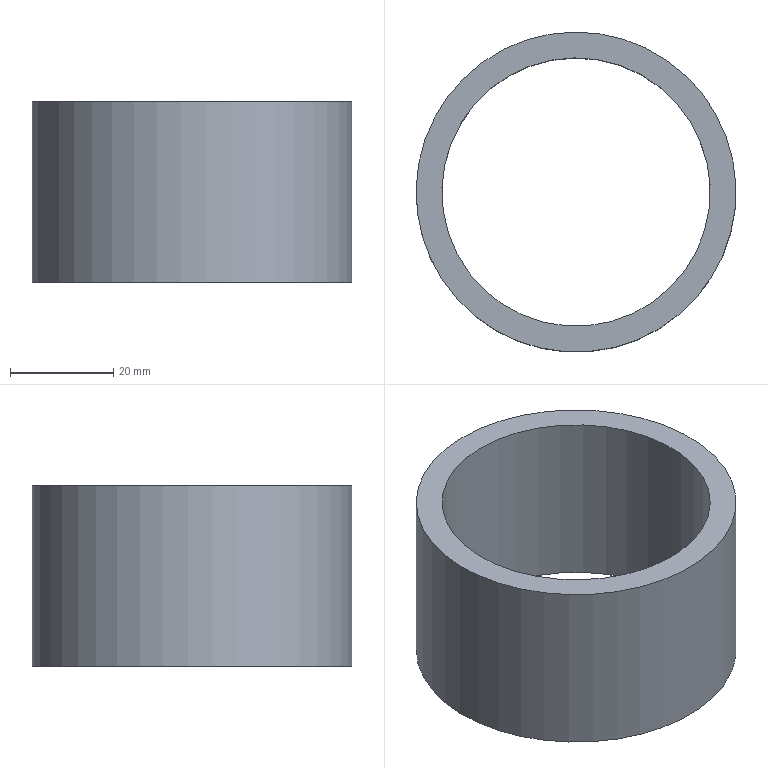Component | NX | CT-ZHOU5-TAOTONG1 | 1 solid | 4 faces | box 62 x 62 x 35 mm | volume 31337 mm3 | cylinder 2 | plane 2 | commonest cylinder face diameters 62 x1 52 x1
STEP:
#1=CARTESIAN_POINT('',(0.,0.,0.));
#2=DIRECTION('',(0.,0.,1.));
#3=DIRECTION('',(1.,0.,0.));
#4=AXIS2_PLACEMENT_3D('',#1,#2,#3);
#5=CARTESIAN_POINT('',(11.875,-28.636,-76.));
#6=VERTEX_POINT('',#5);
#7=CARTESIAN_POINT('',(0.,-0.,-76.));
#8=DIRECTION('',(0.,0.,-1.));
#9=DIRECTION('',(0.383,-0.9237,0.));
#10=AXIS2_PLACEMENT_3D('',#7,#8,#9);
#11=CIRCLE('',#10,31.);
#12=CARTESIAN_POINT('',(0.,-0.,-76.));
#13=DIRECTION('',(0.,0.,1.));
#14=DIRECTION('',(-0.9237,-0.383,0.));
#15=AXIS2_PLACEMENT_3D('',#12,#13,#14);
#16=CYLINDRICAL_SURFACE('',#15,31.);
#17=CARTESIAN_POINT('',(7.854,0.));
#18=DIRECTION('',(-1.,0.));
#19=VECTOR('',#18,1.);
#20=LINE('',#17,#19);
#21=(GEOMETRIC_REPRESENTATION_CONTEXT(2)PARAMETRIC_REPRESENTATION_CONTEXT()REPRESENTATION_CONTEXT('',''));
#22=DEFINITIONAL_REPRESENTATION('',(#20),#21);
#23=PCURVE('',#16,#22);
#24=CARTESIAN_POINT('',(0.,-0.,-76.));
#25=DIRECTION('',(0.,0.,-1.));
#26=DIRECTION('',(0.9237,0.383,0.));
#27=AXIS2_PLACEMENT_3D('',#24,#25,#26);
#28=PLANE('',#27);
#29=CARTESIAN_POINT('',(0.,0.));
#30=DIRECTION('',(0.,1.));
#31=AXIS2_PLACEMENT_2D('',#29,#30);
#32=CIRCLE('',#31,31.);
#33=(GEOMETRIC_REPRESENTATION_CONTEXT(2)PARAMETRIC_REPRESENTATION_CONTEXT()REPRESENTATION_CONTEXT('',''));
#34=DEFINITIONAL_REPRESENTATION('',(#32),#33);
#35=PCURVE('',#28,#34);
#36=SURFACE_CURVE('',#11,(#23,#35),.PCURVE_S1.);
#37=EDGE_CURVE('',#6,#6,#36,.T.);
#38=ORIENTED_EDGE('',*,*,#37,.F.);
#39=CARTESIAN_POINT('',(11.875,-28.636,-41.));
#40=VERTEX_POINT('',#39);
#41=CARTESIAN_POINT('',(11.875,-28.636,-76.));
#42=CARTESIAN_POINT('',(11.875,-28.636,-41.));
#43=B_SPLINE_CURVE_WITH_KNOTS('',1,(#41,#42),.UNSPECIFIED.,.F.,.F.,(2,2),(0.,35.),.PIECEWISE_BEZIER_KNOTS.);
#44=CARTESIAN_POINT('',(7.854,0.));
#45=DIRECTION('',(0.,1.));
#46=VECTOR('',#45,1.);
#47=LINE('',#44,#46);
#48=(GEOMETRIC_REPRESENTATION_CONTEXT(2)PARAMETRIC_REPRESENTATION_CONTEXT()REPRESENTATION_CONTEXT('',''));
#49=DEFINITIONAL_REPRESENTATION('',(#47),#48);
#50=PCURVE('',#16,#49);
#51=CARTESIAN_POINT('',(1.571,0.));
#52=DIRECTION('',(0.,1.));
#53=VECTOR('',#52,1.);
#54=LINE('',#51,#53);
#55=(GEOMETRIC_REPRESENTATION_CONTEXT(2)PARAMETRIC_REPRESENTATION_CONTEXT()REPRESENTATION_CONTEXT('',''));
#56=DEFINITIONAL_REPRESENTATION('',(#54),#55);
#57=PCURVE('',#16,#56);
#58=SEAM_CURVE('',#43,(#50,#57),.PCURVE_S1.);
#59=EDGE_CURVE('',#6,#40,#58,.T.);
#60=ORIENTED_EDGE('',*,*,#59,.T.);
#61=CARTESIAN_POINT('',(0.,-0.,-41.));
#62=DIRECTION('',(0.,0.,-1.));
#63=DIRECTION('',(0.383,-0.9237,0.));
#64=AXIS2_PLACEMENT_3D('',#61,#62,#63);
#65=CIRCLE('',#64,31.);
#66=CARTESIAN_POINT('',(7.854,35.));
#67=DIRECTION('',(-1.,0.));
#68=VECTOR('',#67,1.);
#69=LINE('',#66,#68);
#70=(GEOMETRIC_REPRESENTATION_CONTEXT(2)PARAMETRIC_REPRESENTATION_CONTEXT()REPRESENTATION_CONTEXT('',''));
#71=DEFINITIONAL_REPRESENTATION('',(#69),#70);
#72=PCURVE('',#16,#71);
#73=CARTESIAN_POINT('',(0.,-0.,-41.));
#74=DIRECTION('',(0.,0.,-1.));
#75=DIRECTION('',(0.9237,0.383,0.));
#76=AXIS2_PLACEMENT_3D('',#73,#74,#75);
#77=PLANE('',#76);
#78=CARTESIAN_POINT('',(0.,0.));
#79=DIRECTION('',(0.,1.));
#80=AXIS2_PLACEMENT_2D('',#78,#79);
#81=CIRCLE('',#80,31.);
#82=(GEOMETRIC_REPRESENTATION_CONTEXT(2)PARAMETRIC_REPRESENTATION_CONTEXT()REPRESENTATION_CONTEXT('',''));
#83=DEFINITIONAL_REPRESENTATION('',(#81),#82);
#84=PCURVE('',#77,#83);
#85=SURFACE_CURVE('',#65,(#72,#84),.PCURVE_S1.);
#86=EDGE_CURVE('',#40,#40,#85,.T.);
#87=ORIENTED_EDGE('',*,*,#86,.T.);
#88=ORIENTED_EDGE('',*,*,#59,.F.);
#89=EDGE_LOOP('',(#38,#60,#87,#88));
#90=FACE_BOUND('',#89,.T.);
#91=ADVANCED_FACE('',(#90),#16,.T.);
#92=CARTESIAN_POINT('',(24.017,9.959,-76.));
#93=VERTEX_POINT('',#92);
#94=CARTESIAN_POINT('',(0.,-0.,-76.));
#95=DIRECTION('',(0.,0.,-1.));
#96=DIRECTION('',(0.9237,0.383,0.));
#97=AXIS2_PLACEMENT_3D('',#94,#95,#96);
#98=CIRCLE('',#97,26.);
#99=CARTESIAN_POINT('',(0.,0.));
#100=DIRECTION('',(1.,0.));
#101=AXIS2_PLACEMENT_2D('',#99,#100);
#102=CIRCLE('',#101,26.);
#103=(GEOMETRIC_REPRESENTATION_CONTEXT(2)PARAMETRIC_REPRESENTATION_CONTEXT()REPRESENTATION_CONTEXT('',''));
#104=DEFINITIONAL_REPRESENTATION('',(#102),#103);
#105=PCURVE('',#28,#104);
#106=CARTESIAN_POINT('',(0.,-0.,-40.));
#107=DIRECTION('',(0.,0.,-1.));
#108=DIRECTION('',(0.9237,0.383,0.));
#109=AXIS2_PLACEMENT_3D('',#106,#107,#108);
#110=CYLINDRICAL_SURFACE('',#109,26.);
#111=CARTESIAN_POINT('',(0.,36.));
#112=DIRECTION('',(1.,0.));
#113=VECTOR('',#112,1.);
#114=LINE('',#111,#113);
#115=(GEOMETRIC_REPRESENTATION_CONTEXT(2)PARAMETRIC_REPRESENTATION_CONTEXT()REPRESENTATION_CONTEXT('',''));
#116=DEFINITIONAL_REPRESENTATION('',(#114),#115);
#117=PCURVE('',#110,#116);
#118=SURFACE_CURVE('',#98,(#105,#117),.PCURVE_S1.);
#119=EDGE_CURVE('',#93,#93,#118,.T.);
#120=ORIENTED_EDGE('',*,*,#119,.F.);
#121=EDGE_LOOP('',(#120));
#122=FACE_BOUND('',#121,.T.);
#123=ORIENTED_EDGE('',*,*,#37,.T.);
#124=EDGE_LOOP('',(#123));
#125=FACE_BOUND('',#124,.T.);
#126=ADVANCED_FACE('',(#122,#125),#28,.T.);
#127=CARTESIAN_POINT('',(24.017,9.959,-41.));
#128=VERTEX_POINT('',#127);
#129=CARTESIAN_POINT('',(0.,-0.,-41.));
#130=DIRECTION('',(0.,0.,-1.));
#131=DIRECTION('',(0.9237,0.383,0.));
#132=AXIS2_PLACEMENT_3D('',#129,#130,#131);
#133=CIRCLE('',#132,26.);
#134=CARTESIAN_POINT('',(0.,0.));
#135=DIRECTION('',(1.,0.));
#136=AXIS2_PLACEMENT_2D('',#134,#135);
#137=CIRCLE('',#136,26.);
#138=(GEOMETRIC_REPRESENTATION_CONTEXT(2)PARAMETRIC_REPRESENTATION_CONTEXT()REPRESENTATION_CONTEXT('',''));
#139=DEFINITIONAL_REPRESENTATION('',(#137),#138);
#140=PCURVE('',#77,#139);
#141=CARTESIAN_POINT('',(0.,1.));
#142=DIRECTION('',(1.,0.));
#143=VECTOR('',#142,1.);
#144=LINE('',#141,#143);
#145=(GEOMETRIC_REPRESENTATION_CONTEXT(2)PARAMETRIC_REPRESENTATION_CONTEXT()REPRESENTATION_CONTEXT('',''));
#146=DEFINITIONAL_REPRESENTATION('',(#144),#145);
#147=PCURVE('',#110,#146);
#148=SURFACE_CURVE('',#133,(#140,#147),.PCURVE_S1.);
#149=EDGE_CURVE('',#128,#128,#148,.T.);
#150=ORIENTED_EDGE('',*,*,#149,.T.);
#151=EDGE_LOOP('',(#150));
#152=FACE_BOUND('',#151,.T.);
#153=ORIENTED_EDGE('',*,*,#86,.F.);
#154=EDGE_LOOP('',(#153));
#155=FACE_BOUND('',#154,.T.);
#156=ADVANCED_FACE('',(#152,#155),#77,.F.);
#157=ORIENTED_EDGE('',*,*,#119,.F.);
#158=CARTESIAN_POINT('',(24.017,9.959,-41.));
#159=CARTESIAN_POINT('',(24.017,9.959,-76.));
#160=B_SPLINE_CURVE_WITH_KNOTS('',1,(#158,#159),.UNSPECIFIED.,.F.,.F.,(2,2),(1.,36.),.PIECEWISE_BEZIER_KNOTS.);
#161=CARTESIAN_POINT('',(0.,0.));
#162=DIRECTION('',(0.,1.));
#163=VECTOR('',#162,1.);
#164=LINE('',#161,#163);
#165=(GEOMETRIC_REPRESENTATION_CONTEXT(2)PARAMETRIC_REPRESENTATION_CONTEXT()REPRESENTATION_CONTEXT('',''));
#166=DEFINITIONAL_REPRESENTATION('',(#164),#165);
#167=PCURVE('',#110,#166);
#168=CARTESIAN_POINT('',(6.283,0.));
#169=DIRECTION('',(0.,1.));
#170=VECTOR('',#169,1.);
#171=LINE('',#168,#170);
#172=(GEOMETRIC_REPRESENTATION_CONTEXT(2)PARAMETRIC_REPRESENTATION_CONTEXT()REPRESENTATION_CONTEXT('',''));
#173=DEFINITIONAL_REPRESENTATION('',(#171),#172);
#174=PCURVE('',#110,#173);
#175=SEAM_CURVE('',#160,(#167,#174),.PCURVE_S1.);
#176=EDGE_CURVE('',#128,#93,#175,.T.);
#177=ORIENTED_EDGE('',*,*,#176,.F.);
#178=ORIENTED_EDGE('',*,*,#149,.T.);
#179=ORIENTED_EDGE('',*,*,#176,.T.);
#180=EDGE_LOOP('',(#157,#177,#178,#179));
#181=FACE_BOUND('',#180,.F.);
#182=ADVANCED_FACE('',(#181),#110,.F.);
#183=CLOSED_SHELL('',(#91,#126,#156,#182));
#184=MANIFOLD_SOLID_BREP('',#183);
#185=(LENGTH_UNIT()NAMED_UNIT(*)SI_UNIT(.MILLI.,.METRE.));
#186=UNCERTAINTY_MEASURE_WITH_UNIT(LENGTH_MEASURE(0.00001),#185,'','');
#187=(NAMED_UNIT(*)PLANE_ANGLE_UNIT()SI_UNIT($,.RADIAN.));
#188=(NAMED_UNIT(*)SI_UNIT($,.STERADIAN.)SOLID_ANGLE_UNIT());
#189=(GEOMETRIC_REPRESENTATION_CONTEXT(3)GLOBAL_UNCERTAINTY_ASSIGNED_CONTEXT((#186))GLOBAL_UNIT_ASSIGNED_CONTEXT((#185,#187,#188))REPRESENTATION_CONTEXT('',''));
#190=ADVANCED_BREP_SHAPE_REPRESENTATION('',(#4,#184),#189);